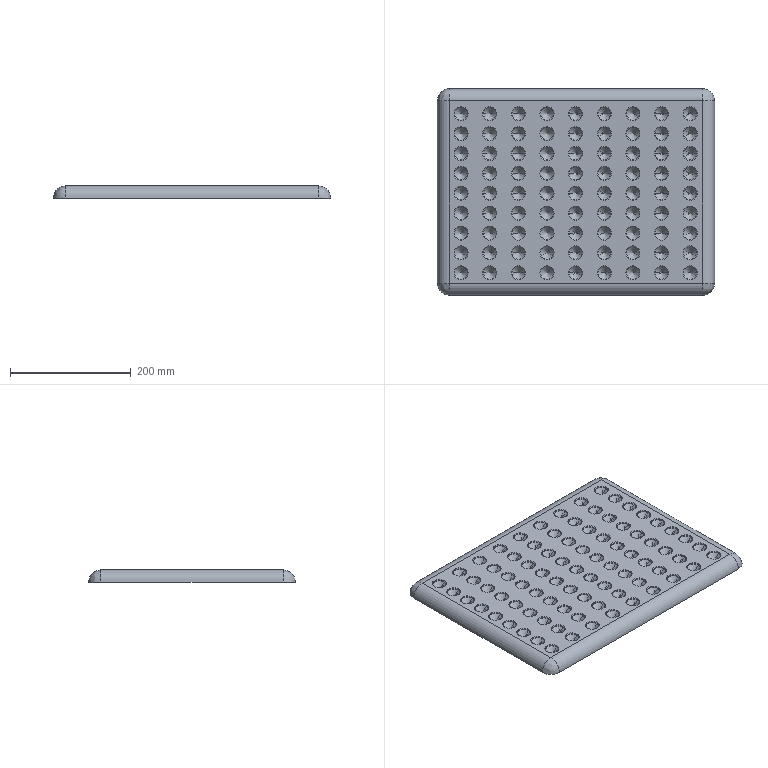Component | SolidWorks | TopPlate-1 | 1 solid | 496 faces | volume 2846644 mm3 | cone 324 | cylinder 166 | spline 4 | plane 2 | commonest cylinder face diameters 21.383 x162 40 x4